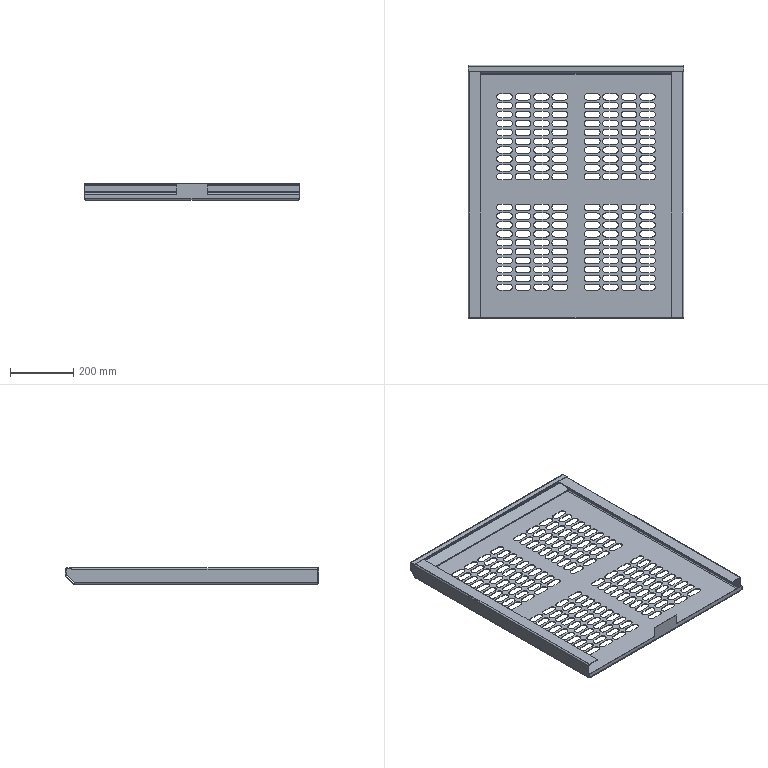Component | NX | SIDE_COVER_PLATE_REAR_LEFT | 1 solid | 712 faces | volume 1154541 mm3 | plane 374 | cylinder 338 | commonest cylinder face diameters 20 x320 6 x10 10 x8